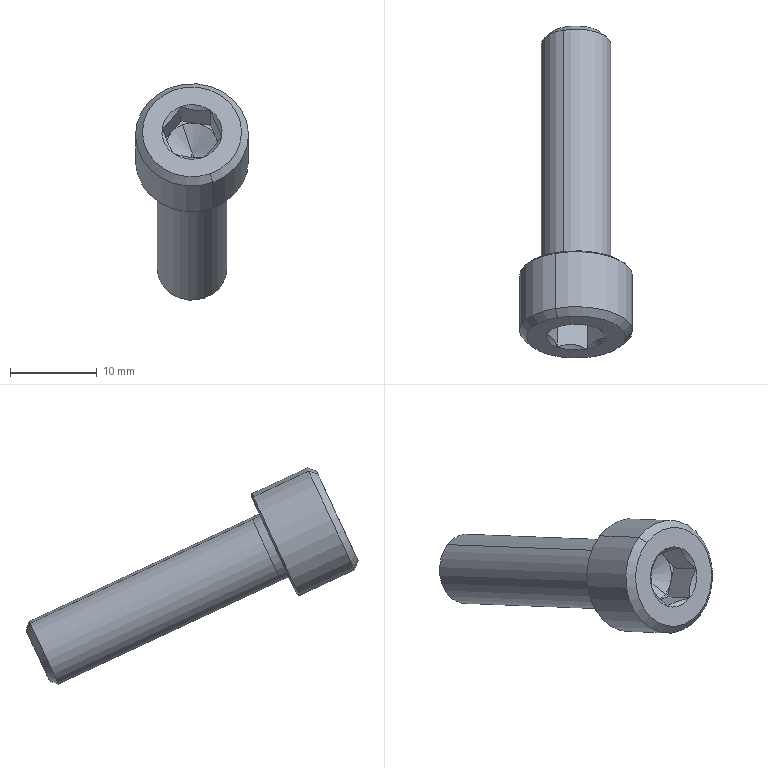Component | SolidWorks | 1369126_DSM_40_270_CC_HD_A_B_0-1_DIN_912_M8x30_F-2 | 1 solid | 35 faces | box 13 x 38.21 x 24.91 mm | volume 2408 mm3 | cone 16 | plane 15 | cylinder 4 | commonest cylinder face diameters 8 x2 13 x2
STEP:
#1=COLOUR_RGB('',0.7922,0.8196,0.9333);
#2=FILL_AREA_STYLE_COLOUR('',#1);
#3=FILL_AREA_STYLE('',(#2));
#4=SURFACE_STYLE_FILL_AREA(#3);
#5=SURFACE_SIDE_STYLE('',(#4));
#6=SURFACE_STYLE_USAGE(.BOTH.,#5);
#7=PRESENTATION_STYLE_ASSIGNMENT((#6));
#8=CARTESIAN_POINT('',(-9.795,80.913,10.266));
#9=VERTEX_POINT('',#8);
#10=CARTESIAN_POINT('',(-9.839,80.898,10.394));
#11=VERTEX_POINT('',#10);
#12=CARTESIAN_POINT('',(-9.839,80.898,10.394));
#13=DIRECTION('',(-0.3195,-0.113,0.9408));
#14=VECTOR('',#13,39.37);
#15=LINE('',#12,#14);
#16=EDGE_CURVE('',#9,#11,#15,.T.);
#17=ORIENTED_EDGE('',*,*,#16,.F.);
#18=CARTESIAN_POINT('',(-9.751,80.805,10.195));
#19=VERTEX_POINT('',#18);
#20=CARTESIAN_POINT('',(-9.751,80.805,10.195));
#21=DIRECTION('',(0.3195,-0.7933,-0.5182));
#22=VECTOR('',#21,39.37);
#23=LINE('',#20,#22);
#24=EDGE_CURVE('',#9,#19,#23,.T.);
#25=ORIENTED_EDGE('',*,*,#24,.T.);
#26=CARTESIAN_POINT('',(-9.702,80.82,10.228));
#27=VERTEX_POINT('',#26);
#28=CARTESIAN_POINT('',(-9.795,80.851,10.295));
#29=DIRECTION('',(0.,-0.9063,0.4226));
#30=DIRECTION('',(-0.3689,0.3928,0.8424));
#31=AXIS2_PLACEMENT_3D('',#28,#29,#30);
#32=CIRCLE('',#31,0.1181);
#33=EDGE_CURVE('',#19,#27,#32,.T.);
#34=ORIENTED_EDGE('',*,*,#33,.T.);
#35=CARTESIAN_POINT('',(-9.685,80.87,10.334));
#36=VERTEX_POINT('',#35);
#37=CARTESIAN_POINT('',(-9.795,80.851,10.295));
#38=DIRECTION('',(0.,-0.9063,0.4226));
#39=DIRECTION('',(-0.3689,0.3928,0.8424));
#40=AXIS2_PLACEMENT_3D('',#37,#38,#39);
#41=CIRCLE('',#40,0.1181);
#42=EDGE_CURVE('',#27,#36,#41,.T.);
#43=ORIENTED_EDGE('',*,*,#42,.T.);
#44=CARTESIAN_POINT('',(-9.778,80.901,10.401));
#45=VERTEX_POINT('',#44);
#46=CARTESIAN_POINT('',(-9.795,80.851,10.295));
#47=DIRECTION('',(0.,-0.9063,0.4226));
#48=DIRECTION('',(-0.3689,0.3928,0.8424));
#49=AXIS2_PLACEMENT_3D('',#46,#47,#48);
#50=CIRCLE('',#49,0.1181);
#51=EDGE_CURVE('',#36,#45,#50,.T.);
#52=ORIENTED_EDGE('',*,*,#51,.T.);
#53=CARTESIAN_POINT('',(-9.795,80.851,10.295));
#54=DIRECTION('',(0.,-0.9063,0.4226));
#55=DIRECTION('',(-0.3689,0.3928,0.8424));
#56=AXIS2_PLACEMENT_3D('',#53,#54,#55);
#57=CIRCLE('',#56,0.1181);
#58=EDGE_CURVE('',#45,#11,#57,.T.);
#59=ORIENTED_EDGE('',*,*,#58,.T.);
#60=EDGE_LOOP('',(#17,#25,#34,#43,#52,#59));
#61=FACE_OUTER_BOUND('',#60,.T.);
#62=CARTESIAN_POINT('',(-9.795,80.851,10.295));
#63=DIRECTION('',(0.,-0.9063,0.4226));
#64=DIRECTION('',(-0.3689,0.3928,0.8424));
#65=AXIS2_PLACEMENT_3D('',#62,#63,#64);
#66=CONICAL_SURFACE('',#65,0.1181,1.047);
#67=ADVANCED_FACE('',(#61),#66,.F.);
#68=CARTESIAN_POINT('',(-9.842,82.114,9.836));
#69=VERTEX_POINT('',#68);
#70=CARTESIAN_POINT('',(-9.748,82.014,9.622));
#71=VERTEX_POINT('',#70);
#72=CARTESIAN_POINT('',(-9.795,82.064,9.729));
#73=DIRECTION('',(0.,-0.9063,0.4226));
#74=DIRECTION('',(-0.3689,0.3928,0.8424));
#75=AXIS2_PLACEMENT_3D('',#72,#73,#74);
#76=CIRCLE('',#75,0.1273);
#77=EDGE_CURVE('',#69,#71,#76,.T.);
#78=ORIENTED_EDGE('',*,*,#77,.T.);
#79=CARTESIAN_POINT('',(-9.737,81.975,9.609));
#80=VERTEX_POINT('',#79);
#81=CARTESIAN_POINT('',(-9.748,82.014,9.622));
#82=DIRECTION('',(0.2609,-0.9186,-0.2968));
#83=VECTOR('',#82,39.37);
#84=LINE('',#81,#83);
#85=EDGE_CURVE('',#71,#80,#84,.T.);
#86=ORIENTED_EDGE('',*,*,#85,.T.);
#87=CARTESIAN_POINT('',(-9.853,82.099,9.874));
#88=VERTEX_POINT('',#87);
#89=CARTESIAN_POINT('',(-9.795,82.037,9.742));
#90=DIRECTION('',(0.,-0.9063,0.4226));
#91=DIRECTION('',(-0.3689,0.3928,0.8424));
#92=AXIS2_PLACEMENT_3D('',#89,#90,#91);
#93=CIRCLE('',#92,0.1575);
#94=EDGE_CURVE('',#88,#80,#93,.T.);
#95=ORIENTED_EDGE('',*,*,#94,.F.);
#96=CARTESIAN_POINT('',(-9.842,82.114,9.836));
#97=DIRECTION('',(-0.2609,-0.3631,0.8945));
#98=VECTOR('',#97,39.37);
#99=LINE('',#96,#98);
#100=EDGE_CURVE('',#69,#88,#99,.T.);
#101=ORIENTED_EDGE('',*,*,#100,.F.);
#102=EDGE_LOOP('',(#78,#86,#95,#101));
#103=FACE_OUTER_BOUND('',#102,.T.);
#104=CARTESIAN_POINT('',(-9.795,82.064,9.729));
#105=DIRECTION('',(0.,-0.9063,0.4226));
#106=DIRECTION('',(-0.3689,0.3928,0.8424));
#107=AXIS2_PLACEMENT_3D('',#104,#105,#106);
#108=CONICAL_SURFACE('',#107,0.1273,0.7854);
#109=ADVANCED_FACE('',(#103),#108,.T.);
#110=ORIENTED_EDGE('',*,*,#94,.T.);
#111=CARTESIAN_POINT('',(-9.737,80.968,10.079));
#112=VERTEX_POINT('',#111);
#113=CARTESIAN_POINT('',(-9.737,82.003,9.596));
#114=DIRECTION('',(0.,-0.9063,0.4226));
#115=VECTOR('',#114,39.37);
#116=LINE('',#113,#115);
#117=EDGE_CURVE('',#80,#112,#116,.T.);
#118=ORIENTED_EDGE('',*,*,#117,.T.);
#119=CARTESIAN_POINT('',(-9.853,81.092,10.344));
#120=VERTEX_POINT('',#119);
#121=CARTESIAN_POINT('',(-9.795,81.03,10.211));
#122=DIRECTION('',(0.,-0.9063,0.4226));
#123=DIRECTION('',(-0.3689,0.3928,0.8424));
#124=AXIS2_PLACEMENT_3D('',#121,#122,#123);
#125=CIRCLE('',#124,0.1575);
#126=EDGE_CURVE('',#120,#112,#125,.T.);
#127=ORIENTED_EDGE('',*,*,#126,.F.);
#128=CARTESIAN_POINT('',(-9.853,82.126,9.862));
#129=DIRECTION('',(0.,-0.9063,0.4226));
#130=VECTOR('',#129,39.37);
#131=LINE('',#128,#130);
#132=EDGE_CURVE('',#88,#120,#131,.T.);
#133=ORIENTED_EDGE('',*,*,#132,.F.);
#134=EDGE_LOOP('',(#110,#118,#127,#133));
#135=FACE_OUTER_BOUND('',#134,.T.);
#136=CARTESIAN_POINT('',(-9.795,82.064,9.729));
#137=DIRECTION('',(0.,-0.9063,0.4226));
#138=DIRECTION('',(-0.3689,0.3928,0.8424));
#139=AXIS2_PLACEMENT_3D('',#136,#137,#138);
#140=CYLINDRICAL_SURFACE('',#139,0.1575);
#141=ADVANCED_FACE('',(#135),#140,.T.);
#142=ORIENTED_EDGE('',*,*,#126,.T.);
#143=CARTESIAN_POINT('',(-9.736,80.931,10.094));
#144=VERTEX_POINT('',#143);
#145=CARTESIAN_POINT('',(-9.737,80.968,10.079));
#146=DIRECTION('',(0.01806,-0.9245,0.3809));
#147=VECTOR('',#146,39.37);
#148=LINE('',#145,#147);
#149=EDGE_CURVE('',#112,#144,#148,.T.);
#150=ORIENTED_EDGE('',*,*,#149,.T.);
#151=CARTESIAN_POINT('',(-9.854,81.057,10.362));
#152=VERTEX_POINT('',#151);
#153=CARTESIAN_POINT('',(-9.795,80.994,10.228));
#154=DIRECTION('',(0.,-0.9063,0.4226));
#155=DIRECTION('',(-0.3689,0.3928,0.8424));
#156=AXIS2_PLACEMENT_3D('',#153,#154,#155);
#157=CIRCLE('',#156,0.1594);
#158=EDGE_CURVE('',#152,#144,#157,.T.);
#159=ORIENTED_EDGE('',*,*,#158,.F.);
#160=CARTESIAN_POINT('',(-9.853,81.092,10.344));
#161=DIRECTION('',(-0.01806,-0.886,0.4634));
#162=VECTOR('',#161,39.37);
#163=LINE('',#160,#162);
#164=EDGE_CURVE('',#120,#152,#163,.T.);
#165=ORIENTED_EDGE('',*,*,#164,.F.);
#166=EDGE_LOOP('',(#142,#150,#159,#165));
#167=FACE_OUTER_BOUND('',#166,.T.);
#168=CARTESIAN_POINT('',(-9.795,81.03,10.211));
#169=DIRECTION('',(0.,-0.9063,0.4226));
#170=DIRECTION('',(-0.3689,0.3928,0.8424));
#171=AXIS2_PLACEMENT_3D('',#168,#169,#170);
#172=CONICAL_SURFACE('',#171,0.1575,0.04898);
#173=ADVANCED_FACE('',(#167),#172,.T.);
#174=CARTESIAN_POINT('',(-9.887,81.091,10.437));
#175=VERTEX_POINT('',#174);
#176=CARTESIAN_POINT('',(-9.703,80.896,10.019));
#177=VERTEX_POINT('',#176);
#178=CARTESIAN_POINT('',(-9.795,80.994,10.228));
#179=DIRECTION('',(0.,-0.9063,0.4226));
#180=DIRECTION('',(-0.3689,0.3928,0.8424));
#181=AXIS2_PLACEMENT_3D('',#178,#179,#180);
#182=CIRCLE('',#181,0.248);
#183=EDGE_CURVE('',#175,#177,#182,.T.);
#184=ORIENTED_EDGE('',*,*,#183,.T.);
#185=CARTESIAN_POINT('',(-9.701,80.886,10.016));
#186=VERTEX_POINT('',#185);
#187=CARTESIAN_POINT('',(-9.703,80.896,10.019));
#188=DIRECTION('',(0.2609,-0.9186,-0.2968));
#189=VECTOR('',#188,39.37);
#190=LINE('',#187,#189);
#191=EDGE_CURVE('',#177,#186,#190,.T.);
#192=ORIENTED_EDGE('',*,*,#191,.T.);
#193=CARTESIAN_POINT('',(-9.889,81.087,10.447));
#194=VERTEX_POINT('',#193);
#195=CARTESIAN_POINT('',(-9.795,80.987,10.232));
#196=DIRECTION('',(0.,-0.9063,0.4226));
#197=DIRECTION('',(-0.3689,0.3928,0.8424));
#198=AXIS2_PLACEMENT_3D('',#195,#196,#197);
#199=CIRCLE('',#198,0.2559);
#200=EDGE_CURVE('',#194,#186,#199,.T.);
#201=ORIENTED_EDGE('',*,*,#200,.F.);
#202=CARTESIAN_POINT('',(-9.887,81.091,10.437));
#203=DIRECTION('',(-0.2609,-0.3631,0.8945));
#204=VECTOR('',#203,39.37);
#205=LINE('',#202,#204);
#206=EDGE_CURVE('',#175,#194,#205,.T.);
#207=ORIENTED_EDGE('',*,*,#206,.F.);
#208=EDGE_LOOP('',(#184,#192,#201,#207));
#209=FACE_OUTER_BOUND('',#208,.T.);
#210=CARTESIAN_POINT('',(-9.795,80.994,10.228));
#211=DIRECTION('',(0.,-0.9063,0.4226));
#212=DIRECTION('',(-0.3689,0.3928,0.8424));
#213=AXIS2_PLACEMENT_3D('',#210,#211,#212);
#214=CONICAL_SURFACE('',#213,0.248,0.7854);
#215=ADVANCED_FACE('',(#209),#214,.T.);
#216=ORIENTED_EDGE('',*,*,#200,.T.);
#217=CARTESIAN_POINT('',(-9.701,80.636,10.132));
#218=VERTEX_POINT('',#217);
#219=CARTESIAN_POINT('',(-9.701,81.964,9.513));
#220=DIRECTION('',(0.,-0.9063,0.4226));
#221=VECTOR('',#220,39.37);
#222=LINE('',#219,#221);
#223=EDGE_CURVE('',#186,#218,#222,.T.);
#224=ORIENTED_EDGE('',*,*,#223,.T.);
#225=CARTESIAN_POINT('',(-9.889,80.838,10.564));
#226=VERTEX_POINT('',#225);
#227=CARTESIAN_POINT('',(-9.795,80.737,10.348));
#228=DIRECTION('',(0.,-0.9063,0.4226));
#229=DIRECTION('',(-0.3689,0.3928,0.8424));
#230=AXIS2_PLACEMENT_3D('',#227,#228,#229);
#231=CIRCLE('',#230,0.2559);
#232=EDGE_CURVE('',#226,#218,#231,.T.);
#233=ORIENTED_EDGE('',*,*,#232,.F.);
#234=CARTESIAN_POINT('',(-9.889,82.165,9.945));
#235=DIRECTION('',(0.,-0.9063,0.4226));
#236=VECTOR('',#235,39.37);
#237=LINE('',#234,#236);
#238=EDGE_CURVE('',#194,#226,#237,.T.);
#239=ORIENTED_EDGE('',*,*,#238,.F.);
#240=EDGE_LOOP('',(#216,#224,#233,#239));
#241=FACE_OUTER_BOUND('',#240,.T.);
#242=CARTESIAN_POINT('',(-9.795,82.064,9.729));
#243=DIRECTION('',(0.,-0.9063,0.4226));
#244=DIRECTION('',(-0.3689,0.3928,0.8424));
#245=AXIS2_PLACEMENT_3D('',#242,#243,#244);
#246=CYLINDRICAL_SURFACE('',#245,0.2559);
#247=ADVANCED_FACE('',(#241),#246,.T.);
#248=CARTESIAN_POINT('',(-9.878,80.797,10.55));
#249=VERTEX_POINT('',#248);
#250=CARTESIAN_POINT('',(-9.712,80.62,10.172));
#251=VERTEX_POINT('',#250);
#252=CARTESIAN_POINT('',(-9.795,80.708,10.361));
#253=DIRECTION('',(0.,-0.9063,0.4226));
#254=DIRECTION('',(-0.3689,0.3928,0.8424));
#255=AXIS2_PLACEMENT_3D('',#252,#253,#254);
#256=CIRCLE('',#255,0.2244);
#257=EDGE_CURVE('',#249,#251,#256,.T.);
#258=ORIENTED_EDGE('',*,*,#257,.F.);
#259=CARTESIAN_POINT('',(-9.889,80.838,10.564));
#260=DIRECTION('',(-0.2609,0.9186,0.2968));
#261=VECTOR('',#260,39.37);
#262=LINE('',#259,#261);
#263=EDGE_CURVE('',#249,#226,#262,.T.);
#264=ORIENTED_EDGE('',*,*,#263,.T.);
#265=ORIENTED_EDGE('',*,*,#232,.T.);
#266=CARTESIAN_POINT('',(-9.701,80.636,10.132));
#267=DIRECTION('',(0.2609,0.3631,-0.8945));
#268=VECTOR('',#267,39.37);
#269=LINE('',#266,#268);
#270=EDGE_CURVE('',#251,#218,#269,.T.);
#271=ORIENTED_EDGE('',*,*,#270,.F.);
#272=EDGE_LOOP('',(#258,#264,#265,#271));
#273=FACE_OUTER_BOUND('',#272,.T.);
#274=CARTESIAN_POINT('',(-9.795,80.737,10.348));
#275=DIRECTION('',(-0.,0.9063,-0.4226));
#276=DIRECTION('',(0.3689,-0.3928,-0.8424));
#277=AXIS2_PLACEMENT_3D('',#274,#275,#276);
#278=CONICAL_SURFACE('',#277,0.2559,0.7854);
#279=ADVANCED_FACE('',(#273),#278,.T.);
#280=CARTESIAN_POINT('',(-9.745,80.655,10.246));
#281=VERTEX_POINT('',#280);
#282=CARTESIAN_POINT('',(-9.66,80.7,10.343));
#283=VERTEX_POINT('',#282);
#284=CARTESIAN_POINT('',(-9.795,80.708,10.361));
#285=DIRECTION('',(0.,-0.9063,0.4226));
#286=DIRECTION('',(-0.3689,0.3928,0.8424));
#287=AXIS2_PLACEMENT_3D('',#284,#285,#286);
#288=CIRCLE('',#287,0.1364);
#289=EDGE_CURVE('',#281,#283,#288,.T.);
#290=ORIENTED_EDGE('',*,*,#289,.T.);
#291=CARTESIAN_POINT('',(-9.66,80.7,10.343));
#292=CARTESIAN_POINT('',(-9.667,80.701,10.334));
#293=CARTESIAN_POINT('',(-9.673,80.702,10.324));
#294=CARTESIAN_POINT('',(-9.684,80.701,10.31));
#295=CARTESIAN_POINT('',(-9.688,80.7,10.305));
#296=CARTESIAN_POINT('',(-9.695,80.698,10.296));
#297=CARTESIAN_POINT('',(-9.699,80.696,10.292));
#298=CARTESIAN_POINT('',(-9.71,80.69,10.279));
#299=CARTESIAN_POINT('',(-9.717,80.685,10.271));
#300=CARTESIAN_POINT('',(-9.731,80.671,10.258));
#301=CARTESIAN_POINT('',(-9.738,80.663,10.252));
#302=CARTESIAN_POINT('',(-9.745,80.655,10.246));
#303=B_SPLINE_CURVE_WITH_KNOTS('',3,(#291,#292,#293,#294,#295,#296,#297,#298,#299,#300,#301,#302),.UNSPECIFIED.,.F.,.F.,(4,2,2,2,2,4),(0.00000025,0.0008948,0.001342,0.001789,0.002684,0.003579),.UNSPECIFIED.);
#304=EDGE_CURVE('',#283,#281,#303,.T.);
#305=ORIENTED_EDGE('',*,*,#304,.T.);
#306=EDGE_LOOP('',(#290,#305));
#307=FACE_OUTER_BOUND('',#306,.T.);
#308=CARTESIAN_POINT('',(-9.795,80.708,10.361));
#309=DIRECTION('',(0.,-0.9063,0.4226));
#310=DIRECTION('',(-0.3689,0.3928,0.8424));
#311=AXIS2_PLACEMENT_3D('',#308,#309,#310);
#312=CONICAL_SURFACE('',#311,0.1364,0.7854);
#313=ADVANCED_FACE('',(#307),#312,.F.);
#314=CARTESIAN_POINT('',(-9.88,80.663,10.264));
#315=VERTEX_POINT('',#314);
#316=CARTESIAN_POINT('',(-9.795,80.708,10.361));
#317=DIRECTION('',(0.,-0.9063,0.4226));
#318=DIRECTION('',(-0.3689,0.3928,0.8424));
#319=AXIS2_PLACEMENT_3D('',#316,#317,#318);
#320=CIRCLE('',#319,0.1364);
#321=EDGE_CURVE('',#315,#281,#320,.T.);
#322=ORIENTED_EDGE('',*,*,#321,.T.);
#323=CARTESIAN_POINT('',(-9.745,80.655,10.246));
#324=CARTESIAN_POINT('',(-9.755,80.66,10.246));
#325=CARTESIAN_POINT('',(-9.766,80.665,10.245));
#326=CARTESIAN_POINT('',(-9.783,80.671,10.245));
#327=CARTESIAN_POINT('',(-9.788,80.672,10.245));
#328=CARTESIAN_POINT('',(-9.8,80.674,10.246));
#329=CARTESIAN_POINT('',(-9.806,80.675,10.247));
#330=CARTESIAN_POINT('',(-9.824,80.676,10.249));
#331=CARTESIAN_POINT('',(-9.835,80.675,10.251));
#332=CARTESIAN_POINT('',(-9.858,80.671,10.257));
#333=CARTESIAN_POINT('',(-9.869,80.667,10.261));
#334=CARTESIAN_POINT('',(-9.88,80.663,10.264));
#335=B_SPLINE_CURVE_WITH_KNOTS('',3,(#323,#324,#325,#326,#327,#328,#329,#330,#331,#332,#333,#334),.UNSPECIFIED.,.F.,.F.,(4,2,2,2,2,4),(0.00000025,0.0008948,0.001342,0.001789,0.002684,0.003579),.UNSPECIFIED.);
#336=EDGE_CURVE('',#281,#315,#335,.T.);
#337=ORIENTED_EDGE('',*,*,#336,.T.);
#338=EDGE_LOOP('',(#322,#337));
#339=FACE_OUTER_BOUND('',#338,.T.);
#340=CARTESIAN_POINT('',(-9.795,80.708,10.361));
#341=DIRECTION('',(0.,-0.9063,0.4226));
#342=DIRECTION('',(-0.3689,0.3928,0.8424));
#343=AXIS2_PLACEMENT_3D('',#340,#341,#342);
#344=CONICAL_SURFACE('',#343,0.1364,0.7854);
#345=ADVANCED_FACE('',(#339),#344,.F.);
#346=CARTESIAN_POINT('',(-9.93,80.717,10.379));
#347=VERTEX_POINT('',#346);
#348=CARTESIAN_POINT('',(-9.795,80.708,10.361));
#349=DIRECTION('',(0.,-0.9063,0.4226));
#350=DIRECTION('',(-0.3689,0.3928,0.8424));
#351=AXIS2_PLACEMENT_3D('',#348,#349,#350);
#352=CIRCLE('',#351,0.1364);
#353=EDGE_CURVE('',#347,#315,#352,.T.);
#354=ORIENTED_EDGE('',*,*,#353,.T.);
#355=CARTESIAN_POINT('',(-9.88,80.663,10.264));
#356=CARTESIAN_POINT('',(-9.884,80.672,10.271));
#357=CARTESIAN_POINT('',(-9.888,80.681,10.278));
#358=CARTESIAN_POINT('',(-9.896,80.696,10.295));
#359=CARTESIAN_POINT('',(-9.9,80.702,10.304));
#360=CARTESIAN_POINT('',(-9.909,80.711,10.324));
#361=CARTESIAN_POINT('',(-9.914,80.714,10.335));
#362=CARTESIAN_POINT('',(-9.92,80.717,10.351));
#363=CARTESIAN_POINT('',(-9.922,80.717,10.357));
#364=CARTESIAN_POINT('',(-9.926,80.717,10.368));
#365=CARTESIAN_POINT('',(-9.928,80.717,10.374));
#366=CARTESIAN_POINT('',(-9.93,80.717,10.379));
#367=B_SPLINE_CURVE_WITH_KNOTS('',3,(#355,#356,#357,#358,#359,#360,#361,#362,#363,#364,#365,#366),.UNSPECIFIED.,.F.,.F.,(4,2,2,2,2,4),(0.00225,0.003148,0.004045,0.004943,0.005392,0.005841),.UNSPECIFIED.);
#368=EDGE_CURVE('',#315,#347,#367,.T.);
#369=ORIENTED_EDGE('',*,*,#368,.T.);
#370=EDGE_LOOP('',(#354,#369));
#371=FACE_OUTER_BOUND('',#370,.T.);
#372=CARTESIAN_POINT('',(-9.795,80.708,10.361));
#373=DIRECTION('',(0.,-0.9063,0.4226));
#374=DIRECTION('',(-0.3689,0.3928,0.8424));
#375=AXIS2_PLACEMENT_3D('',#372,#373,#374);
#376=CONICAL_SURFACE('',#375,0.1364,0.7854);
#377=ADVANCED_FACE('',(#371),#376,.F.);
#378=CARTESIAN_POINT('',(-9.845,80.762,10.476));
#379=VERTEX_POINT('',#378);
#380=CARTESIAN_POINT('',(-9.795,80.708,10.361));
#381=DIRECTION('',(0.,-0.9063,0.4226));
#382=DIRECTION('',(-0.3689,0.3928,0.8424));
#383=AXIS2_PLACEMENT_3D('',#380,#381,#382);
#384=CIRCLE('',#383,0.1364);
#385=EDGE_CURVE('',#379,#347,#384,.T.);
#386=ORIENTED_EDGE('',*,*,#385,.T.);
#387=CARTESIAN_POINT('',(-9.93,80.717,10.379));
#388=CARTESIAN_POINT('',(-9.923,80.725,10.385));
#389=CARTESIAN_POINT('',(-9.917,80.733,10.39));
#390=CARTESIAN_POINT('',(-9.906,80.743,10.4));
#391=CARTESIAN_POINT('',(-9.903,80.746,10.404));
#392=CARTESIAN_POINT('',(-9.895,80.751,10.411));
#393=CARTESIAN_POINT('',(-9.891,80.754,10.416));
#394=CARTESIAN_POINT('',(-9.88,80.76,10.428));
#395=CARTESIAN_POINT('',(-9.873,80.762,10.437));
#396=CARTESIAN_POINT('',(-9.859,80.764,10.457));
#397=CARTESIAN_POINT('',(-9.852,80.763,10.466));
#398=CARTESIAN_POINT('',(-9.845,80.762,10.476));
#399=B_SPLINE_CURVE_WITH_KNOTS('',3,(#387,#388,#389,#390,#391,#392,#393,#394,#395,#396,#397,#398),.UNSPECIFIED.,.F.,.F.,(4,2,2,2,2,4),(0.00000025,0.0008948,0.001342,0.001789,0.002684,0.003579),.UNSPECIFIED.);
#400=EDGE_CURVE('',#347,#379,#399,.T.);
#401=ORIENTED_EDGE('',*,*,#400,.T.);
#402=EDGE_LOOP('',(#386,#401));
#403=FACE_OUTER_BOUND('',#402,.T.);
#404=CARTESIAN_POINT('',(-9.795,80.708,10.361));
#405=DIRECTION('',(0.,-0.9063,0.4226));
#406=DIRECTION('',(-0.3689,0.3928,0.8424));
#407=AXIS2_PLACEMENT_3D('',#404,#405,#406);
#408=CONICAL_SURFACE('',#407,0.1364,0.7854);
#409=ADVANCED_FACE('',(#403),#408,.F.);
#410=CARTESIAN_POINT('',(-9.71,80.754,10.458));
#411=VERTEX_POINT('',#410);
#412=CARTESIAN_POINT('',(-9.795,80.708,10.361));
#413=DIRECTION('',(0.,-0.9063,0.4226));
#414=DIRECTION('',(-0.3689,0.3928,0.8424));
#415=AXIS2_PLACEMENT_3D('',#412,#413,#414);
#416=CIRCLE('',#415,0.1364);
#417=EDGE_CURVE('',#411,#379,#416,.T.);
#418=ORIENTED_EDGE('',*,*,#417,.T.);
#419=CARTESIAN_POINT('',(-9.845,80.762,10.476));
#420=CARTESIAN_POINT('',(-9.835,80.766,10.473));
#421=CARTESIAN_POINT('',(-9.824,80.77,10.469));
#422=CARTESIAN_POINT('',(-9.807,80.773,10.465));
#423=CARTESIAN_POINT('',(-9.802,80.774,10.464));
#424=CARTESIAN_POINT('',(-9.79,80.775,10.461));
#425=CARTESIAN_POINT('',(-9.784,80.775,10.46));
#426=CARTESIAN_POINT('',(-9.766,80.774,10.458));
#427=CARTESIAN_POINT('',(-9.755,80.771,10.457));
#428=CARTESIAN_POINT('',(-9.732,80.764,10.457));
#429=CARTESIAN_POINT('',(-9.721,80.759,10.457));
#430=CARTESIAN_POINT('',(-9.71,80.754,10.458));
#431=B_SPLINE_CURVE_WITH_KNOTS('',3,(#419,#420,#421,#422,#423,#424,#425,#426,#427,#428,#429,#430),.UNSPECIFIED.,.F.,.F.,(4,2,2,2,2,4),(0.00000025,0.0008948,0.001342,0.001789,0.002684,0.003579),.UNSPECIFIED.);
#432=EDGE_CURVE('',#379,#411,#431,.T.);
#433=ORIENTED_EDGE('',*,*,#432,.T.);
#434=EDGE_LOOP('',(#418,#433));
#435=FACE_OUTER_BOUND('',#434,.T.);
#436=CARTESIAN_POINT('',(-9.795,80.708,10.361));
#437=DIRECTION('',(0.,-0.9063,0.4226));
#438=DIRECTION('',(-0.3689,0.3928,0.8424));
#439=AXIS2_PLACEMENT_3D('',#436,#437,#438);
#440=CONICAL_SURFACE('',#439,0.1364,0.7854);
#441=ADVANCED_FACE('',(#435),#440,.F.);
#442=CARTESIAN_POINT('',(-9.795,80.708,10.361));
#443=DIRECTION('',(0.,-0.9063,0.4226));
#444=DIRECTION('',(-0.3689,0.3928,0.8424));
#445=AXIS2_PLACEMENT_3D('',#442,#443,#444);
#446=CIRCLE('',#445,0.1364);
#447=EDGE_CURVE('',#283,#411,#446,.T.);
#448=ORIENTED_EDGE('',*,*,#447,.T.);
#449=CARTESIAN_POINT('',(-9.71,80.754,10.458));
#450=CARTESIAN_POINT('',(-9.708,80.754,10.453));
#451=CARTESIAN_POINT('',(-9.706,80.754,10.447));
#452=CARTESIAN_POINT('',(-9.702,80.754,10.436));
#453=CARTESIAN_POINT('',(-9.7,80.753,10.43));
#454=CARTESIAN_POINT('',(-9.694,80.751,10.414));
#455=CARTESIAN_POINT('',(-9.69,80.748,10.403));
#456=CARTESIAN_POINT('',(-9.681,80.739,10.383));
#457=CARTESIAN_POINT('',(-9.676,80.732,10.374));
#458=CARTESIAN_POINT('',(-9.668,80.718,10.357));
#459=CARTESIAN_POINT('',(-9.664,80.709,10.35));
#460=CARTESIAN_POINT('',(-9.66,80.7,10.343));
#461=B_SPLINE_CURVE_WITH_KNOTS('',3,(#449,#450,#451,#452,#453,#454,#455,#456,#457,#458,#459,#460),.UNSPECIFIED.,.F.,.F.,(4,2,2,2,2,4),(0.001842,0.00229,0.002739,0.003636,0.004533,0.005431),.UNSPECIFIED.);
#462=EDGE_CURVE('',#411,#283,#461,.T.);
#463=ORIENTED_EDGE('',*,*,#462,.T.);
#464=EDGE_LOOP('',(#448,#463));
#465=FACE_OUTER_BOUND('',#464,.T.);
#466=CARTESIAN_POINT('',(-9.795,80.708,10.361));
#467=DIRECTION('',(0.,-0.9063,0.4226));
#468=DIRECTION('',(-0.3689,0.3928,0.8424));
#469=AXIS2_PLACEMENT_3D('',#466,#467,#468);
#470=CONICAL_SURFACE('',#469,0.1364,0.7854);
#471=ADVANCED_FACE('',(#465),#470,.F.);
#472=ORIENTED_EDGE('',*,*,#385,.F.);
#473=ORIENTED_EDGE('',*,*,#417,.F.);
#474=ORIENTED_EDGE('',*,*,#447,.F.);
#475=ORIENTED_EDGE('',*,*,#289,.F.);
#476=ORIENTED_EDGE('',*,*,#321,.F.);
#477=ORIENTED_EDGE('',*,*,#353,.F.);
#478=EDGE_LOOP('',(#472,#473,#474,#475,#476,#477));
#479=FACE_BOUND('',#478,.T.);
#480=CARTESIAN_POINT('',(-9.795,80.708,10.361));
#481=DIRECTION('',(0.,-0.9063,0.4226));
#482=DIRECTION('',(-0.3689,0.3928,0.8424));
#483=AXIS2_PLACEMENT_3D('',#480,#481,#482);
#484=CIRCLE('',#483,0.2244);
#485=EDGE_CURVE('',#251,#249,#484,.T.);
#486=ORIENTED_EDGE('',*,*,#485,.T.);
#487=ORIENTED_EDGE('',*,*,#257,.T.);
#488=EDGE_LOOP('',(#486,#487));
#489=FACE_OUTER_BOUND('',#488,.T.);
#490=CARTESIAN_POINT('',(-9.922,80.687,10.316));
#491=DIRECTION('',(-0.,0.9063,-0.4226));
#492=DIRECTION('',(0.3689,-0.3928,-0.8424));
#493=AXIS2_PLACEMENT_3D('',#490,#491,#492);
#494=PLANE('',#493);
#495=ADVANCED_FACE('',(#479,#489),#494,.F.);
#496=ORIENTED_EDGE('',*,*,#263,.F.);
#497=ORIENTED_EDGE('',*,*,#485,.F.);
#498=ORIENTED_EDGE('',*,*,#270,.T.);
#499=CARTESIAN_POINT('',(-9.795,80.737,10.348));
#500=DIRECTION('',(0.,-0.9063,0.4226));
#501=DIRECTION('',(-0.3689,0.3928,0.8424));
#502=AXIS2_PLACEMENT_3D('',#499,#500,#501);
#503=CIRCLE('',#502,0.2559);
#504=EDGE_CURVE('',#218,#226,#503,.T.);
#505=ORIENTED_EDGE('',*,*,#504,.T.);
#506=EDGE_LOOP('',(#496,#497,#498,#505));
#507=FACE_OUTER_BOUND('',#506,.T.);
#508=CARTESIAN_POINT('',(-9.795,80.737,10.348));
#509=DIRECTION('',(-0.,0.9063,-0.4226));
#510=DIRECTION('',(0.3689,-0.3928,-0.8424));
#511=AXIS2_PLACEMENT_3D('',#508,#509,#510);
#512=CONICAL_SURFACE('',#511,0.2559,0.7854);
#513=ADVANCED_FACE('',(#507),#512,.T.);
#514=ORIENTED_EDGE('',*,*,#223,.F.);
#515=CARTESIAN_POINT('',(-9.795,80.987,10.232));
#516=DIRECTION('',(0.,-0.9063,0.4226));
#517=DIRECTION('',(-0.3689,0.3928,0.8424));
#518=AXIS2_PLACEMENT_3D('',#515,#516,#517);
#519=CIRCLE('',#518,0.2559);
#520=EDGE_CURVE('',#186,#194,#519,.T.);
#521=ORIENTED_EDGE('',*,*,#520,.T.);
#522=ORIENTED_EDGE('',*,*,#238,.T.);
#523=ORIENTED_EDGE('',*,*,#504,.F.);
#524=EDGE_LOOP('',(#514,#521,#522,#523));
#525=FACE_OUTER_BOUND('',#524,.T.);
#526=CARTESIAN_POINT('',(-9.795,82.064,9.729));
#527=DIRECTION('',(0.,-0.9063,0.4226));
#528=DIRECTION('',(-0.3689,0.3928,0.8424));
#529=AXIS2_PLACEMENT_3D('',#526,#527,#528);
#530=CYLINDRICAL_SURFACE('',#529,0.2559);
#531=ADVANCED_FACE('',(#525),#530,.T.);
#532=ORIENTED_EDGE('',*,*,#191,.F.);
#533=CARTESIAN_POINT('',(-9.795,80.994,10.228));
#534=DIRECTION('',(0.,-0.9063,0.4226));
#535=DIRECTION('',(-0.3689,0.3928,0.8424));
#536=AXIS2_PLACEMENT_3D('',#533,#534,#535);
#537=CIRCLE('',#536,0.248);
#538=EDGE_CURVE('',#177,#175,#537,.T.);
#539=ORIENTED_EDGE('',*,*,#538,.T.);
#540=ORIENTED_EDGE('',*,*,#206,.T.);
#541=ORIENTED_EDGE('',*,*,#520,.F.);
#542=EDGE_LOOP('',(#532,#539,#540,#541));
#543=FACE_OUTER_BOUND('',#542,.T.);
#544=CARTESIAN_POINT('',(-9.795,80.994,10.228));
#545=DIRECTION('',(0.,-0.9063,0.4226));
#546=DIRECTION('',(-0.3689,0.3928,0.8424));
#547=AXIS2_PLACEMENT_3D('',#544,#545,#546);
#548=CONICAL_SURFACE('',#547,0.248,0.7854);
#549=ADVANCED_FACE('',(#543),#548,.T.);
#550=ORIENTED_EDGE('',*,*,#183,.F.);
#551=ORIENTED_EDGE('',*,*,#538,.F.);
#552=EDGE_LOOP('',(#550,#551));
#553=FACE_OUTER_BOUND('',#552,.T.);
#554=ORIENTED_EDGE('',*,*,#158,.T.);
#555=CARTESIAN_POINT('',(-9.795,80.994,10.228));
#556=DIRECTION('',(0.,-0.9063,0.4226));
#557=DIRECTION('',(-0.3689,0.3928,0.8424));
#558=AXIS2_PLACEMENT_3D('',#555,#556,#557);
#559=CIRCLE('',#558,0.1594);
#560=EDGE_CURVE('',#144,#152,#559,.T.);
#561=ORIENTED_EDGE('',*,*,#560,.T.);
#562=EDGE_LOOP('',(#554,#561));
#563=FACE_BOUND('',#562,.T.);
#564=CARTESIAN_POINT('',(-10.026,80.955,10.145));
#565=DIRECTION('',(0.,-0.9063,0.4226));
#566=DIRECTION('',(-0.3689,0.3928,0.8424));
#567=AXIS2_PLACEMENT_3D('',#564,#565,#566);
#568=PLANE('',#567);
#569=ADVANCED_FACE('',(#553,#563),#568,.F.);
#570=ORIENTED_EDGE('',*,*,#149,.F.);
#571=CARTESIAN_POINT('',(-9.795,81.03,10.211));
#572=DIRECTION('',(0.,-0.9063,0.4226));
#573=DIRECTION('',(-0.3689,0.3928,0.8424));
#574=AXIS2_PLACEMENT_3D('',#571,#572,#573);
#575=CIRCLE('',#574,0.1575);
#576=EDGE_CURVE('',#112,#120,#575,.T.);
#577=ORIENTED_EDGE('',*,*,#576,.T.);
#578=ORIENTED_EDGE('',*,*,#164,.T.);
#579=ORIENTED_EDGE('',*,*,#560,.F.);
#580=EDGE_LOOP('',(#570,#577,#578,#579));
#581=FACE_OUTER_BOUND('',#580,.T.);
#582=CARTESIAN_POINT('',(-9.795,81.03,10.211));
#583=DIRECTION('',(0.,-0.9063,0.4226));
#584=DIRECTION('',(-0.3689,0.3928,0.8424));
#585=AXIS2_PLACEMENT_3D('',#582,#583,#584);
#586=CONICAL_SURFACE('',#585,0.1575,0.04898);
#587=ADVANCED_FACE('',(#581),#586,.T.);
#588=ORIENTED_EDGE('',*,*,#117,.F.);
#589=CARTESIAN_POINT('',(-9.795,82.037,9.742));
#590=DIRECTION('',(0.,-0.9063,0.4226));
#591=DIRECTION('',(-0.3689,0.3928,0.8424));
#592=AXIS2_PLACEMENT_3D('',#589,#590,#591);
#593=CIRCLE('',#592,0.1575);
#594=EDGE_CURVE('',#80,#88,#593,.T.);
#595=ORIENTED_EDGE('',*,*,#594,.T.);
#596=ORIENTED_EDGE('',*,*,#132,.T.);
#597=ORIENTED_EDGE('',*,*,#576,.F.);
#598=EDGE_LOOP('',(#588,#595,#596,#597));
#599=FACE_OUTER_BOUND('',#598,.T.);
#600=CARTESIAN_POINT('',(-9.795,82.064,9.729));
#601=DIRECTION('',(0.,-0.9063,0.4226));
#602=DIRECTION('',(-0.3689,0.3928,0.8424));
#603=AXIS2_PLACEMENT_3D('',#600,#601,#602);
#604=CYLINDRICAL_SURFACE('',#603,0.1575);
#605=ADVANCED_FACE('',(#599),#604,.T.);
#606=ORIENTED_EDGE('',*,*,#85,.F.);
#607=CARTESIAN_POINT('',(-9.795,82.064,9.729));
#608=DIRECTION('',(0.,-0.9063,0.4226));
#609=DIRECTION('',(-0.3689,0.3928,0.8424));
#610=AXIS2_PLACEMENT_3D('',#607,#608,#609);
#611=CIRCLE('',#610,0.1273);
#612=EDGE_CURVE('',#71,#69,#611,.T.);
#613=ORIENTED_EDGE('',*,*,#612,.T.);
#614=ORIENTED_EDGE('',*,*,#100,.T.);
#615=ORIENTED_EDGE('',*,*,#594,.F.);
#616=EDGE_LOOP('',(#606,#613,#614,#615));
#617=FACE_OUTER_BOUND('',#616,.T.);
#618=CARTESIAN_POINT('',(-9.795,82.064,9.729));
#619=DIRECTION('',(0.,-0.9063,0.4226));
#620=DIRECTION('',(-0.3689,0.3928,0.8424));
#621=AXIS2_PLACEMENT_3D('',#618,#619,#620);
#622=CONICAL_SURFACE('',#621,0.1273,0.7854);
#623=ADVANCED_FACE('',(#617),#622,.T.);
#624=ORIENTED_EDGE('',*,*,#77,.F.);
#625=ORIENTED_EDGE('',*,*,#612,.F.);
#626=EDGE_LOOP('',(#624,#625));
#627=FACE_OUTER_BOUND('',#626,.T.);
#628=CARTESIAN_POINT('',(-9.913,82.045,9.686));
#629=DIRECTION('',(0.,-0.9063,0.4226));
#630=DIRECTION('',(-0.3689,0.3928,0.8424));
#631=AXIS2_PLACEMENT_3D('',#628,#629,#630);
#632=PLANE('',#631);
#633=ADVANCED_FACE('',(#627),#632,.F.);
#634=ORIENTED_EDGE('',*,*,#51,.F.);
#635=CARTESIAN_POINT('',(-9.71,80.896,10.392));
#636=VERTEX_POINT('',#635);
#637=CARTESIAN_POINT('',(-9.66,80.843,10.277));
#638=DIRECTION('',(-0.3689,0.3928,0.8424));
#639=VECTOR('',#638,39.37);
#640=LINE('',#637,#639);
#641=EDGE_CURVE('',#36,#636,#640,.T.);
#642=ORIENTED_EDGE('',*,*,#641,.T.);
#643=CARTESIAN_POINT('',(-9.71,80.896,10.392));
#644=DIRECTION('',(-0.9894,0.06137,0.1316));
#645=VECTOR('',#644,39.37);
#646=LINE('',#643,#645);
#647=EDGE_CURVE('',#636,#45,#646,.T.);
#648=ORIENTED_EDGE('',*,*,#647,.T.);
#649=EDGE_LOOP('',(#634,#642,#648));
#650=FACE_OUTER_BOUND('',#649,.T.);
#651=CARTESIAN_POINT('',(-9.795,80.851,10.295));
#652=DIRECTION('',(0.,-0.9063,0.4226));
#653=DIRECTION('',(-0.3689,0.3928,0.8424));
#654=AXIS2_PLACEMENT_3D('',#651,#652,#653);
#655=PLANE('',#654);
#656=ADVANCED_FACE('',(#650),#655,.T.);
#657=ORIENTED_EDGE('',*,*,#42,.F.);
#658=CARTESIAN_POINT('',(-9.66,80.843,10.277));
#659=VERTEX_POINT('',#658);
#660=CARTESIAN_POINT('',(-9.745,80.798,10.18));
#661=DIRECTION('',(0.6205,0.3314,0.7108));
#662=VECTOR('',#661,39.37);
#663=LINE('',#660,#662);
#664=EDGE_CURVE('',#27,#659,#663,.T.);
#665=ORIENTED_EDGE('',*,*,#664,.T.);
#666=CARTESIAN_POINT('',(-9.66,80.843,10.277));
#667=DIRECTION('',(-0.3689,0.3928,0.8424));
#668=VECTOR('',#667,39.37);
#669=LINE('',#666,#668);
#670=EDGE_CURVE('',#659,#36,#669,.T.);
#671=ORIENTED_EDGE('',*,*,#670,.T.);
#672=EDGE_LOOP('',(#657,#665,#671));
#673=FACE_OUTER_BOUND('',#672,.T.);
#674=CARTESIAN_POINT('',(-9.795,80.851,10.295));
#675=DIRECTION('',(0.,-0.9063,0.4226));
#676=DIRECTION('',(-0.3689,0.3928,0.8424));
#677=AXIS2_PLACEMENT_3D('',#674,#675,#676);
#678=PLANE('',#677);
#679=ADVANCED_FACE('',(#673),#678,.T.);
#680=CARTESIAN_POINT('',(-9.812,80.802,10.189));
#681=VERTEX_POINT('',#680);
#682=CARTESIAN_POINT('',(-9.795,80.851,10.295));
#683=DIRECTION('',(0.,-0.9063,0.4226));
#684=DIRECTION('',(-0.3689,0.3928,0.8424));
#685=AXIS2_PLACEMENT_3D('',#682,#683,#684);
#686=CIRCLE('',#685,0.1181);
#687=EDGE_CURVE('',#681,#19,#686,.T.);
#688=ORIENTED_EDGE('',*,*,#687,.F.);
#689=CARTESIAN_POINT('',(-9.745,80.798,10.18));
#690=VERTEX_POINT('',#689);
#691=CARTESIAN_POINT('',(-9.88,80.806,10.198));
#692=DIRECTION('',(0.9894,-0.06137,-0.1316));
#693=VECTOR('',#692,39.37);
#694=LINE('',#691,#693);
#695=EDGE_CURVE('',#681,#690,#694,.T.);
#696=ORIENTED_EDGE('',*,*,#695,.T.);
#697=CARTESIAN_POINT('',(-9.745,80.798,10.18));
#698=DIRECTION('',(0.6205,0.3314,0.7108));
#699=VECTOR('',#698,39.37);
#700=LINE('',#697,#699);
#701=EDGE_CURVE('',#690,#27,#700,.T.);
#702=ORIENTED_EDGE('',*,*,#701,.T.);
#703=ORIENTED_EDGE('',*,*,#33,.F.);
#704=EDGE_LOOP('',(#688,#696,#702,#703));
#705=FACE_OUTER_BOUND('',#704,.T.);
#706=CARTESIAN_POINT('',(-9.795,80.851,10.295));
#707=DIRECTION('',(0.,-0.9063,0.4226));
#708=DIRECTION('',(-0.3689,0.3928,0.8424));
#709=AXIS2_PLACEMENT_3D('',#706,#707,#708);
#710=PLANE('',#709);
#711=ADVANCED_FACE('',(#705),#710,.T.);
#712=CARTESIAN_POINT('',(-9.905,80.833,10.255));
#713=VERTEX_POINT('',#712);
#714=CARTESIAN_POINT('',(-9.795,80.851,10.295));
#715=DIRECTION('',(0.,-0.9063,0.4226));
#716=DIRECTION('',(-0.3689,0.3928,0.8424));
#717=AXIS2_PLACEMENT_3D('',#714,#715,#716);
#718=CIRCLE('',#717,0.1181);
#719=EDGE_CURVE('',#713,#681,#718,.T.);
#720=ORIENTED_EDGE('',*,*,#719,.F.);
#721=CARTESIAN_POINT('',(-9.88,80.806,10.198));
#722=VERTEX_POINT('',#721);
#723=CARTESIAN_POINT('',(-9.93,80.86,10.313));
#724=DIRECTION('',(0.3689,-0.3928,-0.8424));
#725=VECTOR('',#724,39.37);
#726=LINE('',#723,#725);
#727=EDGE_CURVE('',#713,#722,#726,.T.);
#728=ORIENTED_EDGE('',*,*,#727,.T.);
#729=CARTESIAN_POINT('',(-9.88,80.806,10.198));
#730=DIRECTION('',(0.9894,-0.06137,-0.1316));
#731=VECTOR('',#730,39.37);
#732=LINE('',#729,#731);
#733=EDGE_CURVE('',#722,#681,#732,.T.);
#734=ORIENTED_EDGE('',*,*,#733,.T.);
#735=EDGE_LOOP('',(#720,#728,#734));
#736=FACE_OUTER_BOUND('',#735,.T.);
#737=CARTESIAN_POINT('',(-9.795,80.851,10.295));
#738=DIRECTION('',(0.,-0.9063,0.4226));
#739=DIRECTION('',(-0.3689,0.3928,0.8424));
#740=AXIS2_PLACEMENT_3D('',#737,#738,#739);
#741=PLANE('',#740);
#742=ADVANCED_FACE('',(#736),#741,.T.);
#743=CARTESIAN_POINT('',(-9.888,80.882,10.361));
#744=VERTEX_POINT('',#743);
#745=CARTESIAN_POINT('',(-9.795,80.851,10.295));
#746=DIRECTION('',(0.,-0.9063,0.4226));
#747=DIRECTION('',(-0.3689,0.3928,0.8424));
#748=AXIS2_PLACEMENT_3D('',#745,#746,#747);
#749=CIRCLE('',#748,0.1181);
#750=EDGE_CURVE('',#744,#713,#749,.T.);
#751=ORIENTED_EDGE('',*,*,#750,.F.);
#752=CARTESIAN_POINT('',(-9.93,80.86,10.313));
#753=VERTEX_POINT('',#752);
#754=CARTESIAN_POINT('',(-9.845,80.905,10.41));
#755=DIRECTION('',(-0.6205,-0.3314,-0.7108));
#756=VECTOR('',#755,39.37);
#757=LINE('',#754,#756);
#758=EDGE_CURVE('',#744,#753,#757,.T.);
#759=ORIENTED_EDGE('',*,*,#758,.T.);
#760=CARTESIAN_POINT('',(-9.93,80.86,10.313));
#761=DIRECTION('',(0.3689,-0.3928,-0.8424));
#762=VECTOR('',#761,39.37);
#763=LINE('',#760,#762);
#764=EDGE_CURVE('',#753,#713,#763,.T.);
#765=ORIENTED_EDGE('',*,*,#764,.T.);
#766=EDGE_LOOP('',(#751,#759,#765));
#767=FACE_OUTER_BOUND('',#766,.T.);
#768=CARTESIAN_POINT('',(-9.795,80.851,10.295));
#769=DIRECTION('',(0.,-0.9063,0.4226));
#770=DIRECTION('',(-0.3689,0.3928,0.8424));
#771=AXIS2_PLACEMENT_3D('',#768,#769,#770);
#772=PLANE('',#771);
#773=ADVANCED_FACE('',(#767),#772,.T.);
#774=ORIENTED_EDGE('',*,*,#58,.F.);
#775=CARTESIAN_POINT('',(-9.845,80.905,10.41));
#776=VERTEX_POINT('',#775);
#777=CARTESIAN_POINT('',(-9.71,80.896,10.392));
#778=DIRECTION('',(-0.9894,0.06137,0.1316));
#779=VECTOR('',#778,39.37);
#780=LINE('',#777,#779);
#781=EDGE_CURVE('',#45,#776,#780,.T.);
#782=ORIENTED_EDGE('',*,*,#781,.T.);
#783=CARTESIAN_POINT('',(-9.845,80.905,10.41));
#784=DIRECTION('',(-0.6205,-0.3314,-0.7108));
#785=VECTOR('',#784,39.37);
#786=LINE('',#783,#785);
#787=EDGE_CURVE('',#776,#744,#786,.T.);
#788=ORIENTED_EDGE('',*,*,#787,.T.);
#789=CARTESIAN_POINT('',(-9.795,80.851,10.295));
#790=DIRECTION('',(0.,-0.9063,0.4226));
#791=DIRECTION('',(-0.3689,0.3928,0.8424));
#792=AXIS2_PLACEMENT_3D('',#789,#790,#791);
#793=CIRCLE('',#792,0.1181);
#794=EDGE_CURVE('',#11,#744,#793,.T.);
#795=ORIENTED_EDGE('',*,*,#794,.F.);
#796=EDGE_LOOP('',(#774,#782,#788,#795));
#797=FACE_OUTER_BOUND('',#796,.T.);
#798=CARTESIAN_POINT('',(-9.795,80.851,10.295));
#799=DIRECTION('',(0.,-0.9063,0.4226));
#800=DIRECTION('',(-0.3689,0.3928,0.8424));
#801=AXIS2_PLACEMENT_3D('',#798,#799,#800);
#802=PLANE('',#801);
#803=ADVANCED_FACE('',(#797),#802,.T.);
#804=ORIENTED_EDGE('',*,*,#304,.F.);
#805=CARTESIAN_POINT('',(-9.66,80.843,10.277));
#806=DIRECTION('',(0.,-0.9063,0.4226));
#807=VECTOR('',#806,39.37);
#808=LINE('',#805,#807);
#809=EDGE_CURVE('',#659,#283,#808,.T.);
#810=ORIENTED_EDGE('',*,*,#809,.F.);
#811=ORIENTED_EDGE('',*,*,#664,.F.);
#812=ORIENTED_EDGE('',*,*,#701,.F.);
#813=CARTESIAN_POINT('',(-9.745,80.798,10.18));
#814=DIRECTION('',(0.,-0.9063,0.4226));
#815=VECTOR('',#814,39.37);
#816=LINE('',#813,#815);
#817=EDGE_CURVE('',#690,#281,#816,.T.);
#818=ORIENTED_EDGE('',*,*,#817,.T.);
#819=EDGE_LOOP('',(#804,#810,#811,#812,#818));
#820=FACE_OUTER_BOUND('',#819,.T.);
#821=CARTESIAN_POINT('',(-9.745,80.798,10.18));
#822=DIRECTION('',(0.7842,-0.2622,-0.5623));
#823=DIRECTION('',(0.6205,0.3314,0.7108));
#824=AXIS2_PLACEMENT_3D('',#821,#822,#823);
#825=PLANE('',#824);
#826=ADVANCED_FACE('',(#820),#825,.F.);
#827=ORIENTED_EDGE('',*,*,#336,.F.);
#828=ORIENTED_EDGE('',*,*,#817,.F.);
#829=ORIENTED_EDGE('',*,*,#695,.F.);
#830=ORIENTED_EDGE('',*,*,#733,.F.);
#831=CARTESIAN_POINT('',(-9.88,80.806,10.198));
#832=DIRECTION('',(0.,-0.9063,0.4226));
#833=VECTOR('',#832,39.37);
#834=LINE('',#831,#833);
#835=EDGE_CURVE('',#722,#315,#834,.T.);
#836=ORIENTED_EDGE('',*,*,#835,.T.);
#837=EDGE_LOOP('',(#827,#828,#829,#830,#836));
#838=FACE_OUTER_BOUND('',#837,.T.);
#839=CARTESIAN_POINT('',(-9.88,80.806,10.198));
#840=DIRECTION('',(-0.1452,-0.4181,-0.8967));
#841=DIRECTION('',(0.9894,-0.06137,-0.1316));
#842=AXIS2_PLACEMENT_3D('',#839,#840,#841);
#843=PLANE('',#842);
#844=ADVANCED_FACE('',(#838),#843,.F.);
#845=ORIENTED_EDGE('',*,*,#368,.F.);
#846=ORIENTED_EDGE('',*,*,#835,.F.);
#847=ORIENTED_EDGE('',*,*,#727,.F.);
#848=ORIENTED_EDGE('',*,*,#764,.F.);
#849=CARTESIAN_POINT('',(-9.93,80.86,10.313));
#850=DIRECTION('',(0.,-0.9063,0.4226));
#851=VECTOR('',#850,39.37);
#852=LINE('',#849,#851);
#853=EDGE_CURVE('',#753,#347,#852,.T.);
#854=ORIENTED_EDGE('',*,*,#853,.T.);
#855=EDGE_LOOP('',(#845,#846,#847,#848,#854));
#856=FACE_OUTER_BOUND('',#855,.T.);
#857=CARTESIAN_POINT('',(-9.93,80.86,10.313));
#858=DIRECTION('',(-0.9295,-0.1559,-0.3344));
#859=DIRECTION('',(0.3689,-0.3928,-0.8424));
#860=AXIS2_PLACEMENT_3D('',#857,#858,#859);
#861=PLANE('',#860);
#862=ADVANCED_FACE('',(#856),#861,.F.);
#863=ORIENTED_EDGE('',*,*,#400,.F.);
#864=ORIENTED_EDGE('',*,*,#853,.F.);
#865=ORIENTED_EDGE('',*,*,#758,.F.);
#866=ORIENTED_EDGE('',*,*,#787,.F.);
#867=CARTESIAN_POINT('',(-9.845,80.905,10.41));
#868=DIRECTION('',(0.,-0.9063,0.4226));
#869=VECTOR('',#868,39.37);
#870=LINE('',#867,#869);
#871=EDGE_CURVE('',#776,#379,#870,.T.);
#872=ORIENTED_EDGE('',*,*,#871,.T.);
#873=EDGE_LOOP('',(#863,#864,#865,#866,#872));
#874=FACE_OUTER_BOUND('',#873,.T.);
#875=CARTESIAN_POINT('',(-9.845,80.905,10.41));
#876=DIRECTION('',(-0.7842,0.2622,0.5623));
#877=DIRECTION('',(-0.6205,-0.3314,-0.7108));
#878=AXIS2_PLACEMENT_3D('',#875,#876,#877);
#879=PLANE('',#878);
#880=ADVANCED_FACE('',(#874),#879,.F.);
#881=ORIENTED_EDGE('',*,*,#432,.F.);
#882=ORIENTED_EDGE('',*,*,#871,.F.);
#883=ORIENTED_EDGE('',*,*,#781,.F.);
#884=ORIENTED_EDGE('',*,*,#647,.F.);
#885=CARTESIAN_POINT('',(-9.71,80.896,10.392));
#886=DIRECTION('',(0.,-0.9063,0.4226));
#887=VECTOR('',#886,39.37);
#888=LINE('',#885,#887);
#889=EDGE_CURVE('',#636,#411,#888,.T.);
#890=ORIENTED_EDGE('',*,*,#889,.T.);
#891=EDGE_LOOP('',(#881,#882,#883,#884,#890));
#892=FACE_OUTER_BOUND('',#891,.T.);
#893=CARTESIAN_POINT('',(-9.71,80.896,10.392));
#894=DIRECTION('',(0.1452,0.4181,0.8967));
#895=DIRECTION('',(-0.9894,0.06137,0.1316));
#896=AXIS2_PLACEMENT_3D('',#893,#894,#895);
#897=PLANE('',#896);
#898=ADVANCED_FACE('',(#892),#897,.F.);
#899=ORIENTED_EDGE('',*,*,#462,.F.);
#900=ORIENTED_EDGE('',*,*,#889,.F.);
#901=ORIENTED_EDGE('',*,*,#641,.F.);
#902=ORIENTED_EDGE('',*,*,#670,.F.);
#903=ORIENTED_EDGE('',*,*,#809,.T.);
#904=EDGE_LOOP('',(#899,#900,#901,#902,#903));
#905=FACE_OUTER_BOUND('',#904,.T.);
#906=CARTESIAN_POINT('',(-9.66,80.843,10.277));
#907=DIRECTION('',(0.9295,0.1559,0.3344));
#908=DIRECTION('',(-0.3689,0.3928,0.8424));
#909=AXIS2_PLACEMENT_3D('',#906,#907,#908);
#910=PLANE('',#909);
#911=ADVANCED_FACE('',(#905),#910,.F.);
#912=ORIENTED_EDGE('',*,*,#24,.F.);
#913=ORIENTED_EDGE('',*,*,#16,.T.);
#914=ORIENTED_EDGE('',*,*,#794,.T.);
#915=ORIENTED_EDGE('',*,*,#750,.T.);
#916=ORIENTED_EDGE('',*,*,#719,.T.);
#917=ORIENTED_EDGE('',*,*,#687,.T.);
#918=EDGE_LOOP('',(#912,#913,#914,#915,#916,#917));
#919=FACE_OUTER_BOUND('',#918,.T.);
#920=CARTESIAN_POINT('',(-9.795,80.851,10.295));
#921=DIRECTION('',(0.,-0.9063,0.4226));
#922=DIRECTION('',(-0.3689,0.3928,0.8424));
#923=AXIS2_PLACEMENT_3D('',#920,#921,#922);
#924=CONICAL_SURFACE('',#923,0.1181,1.047);
#925=ADVANCED_FACE('',(#919),#924,.F.);
#926=CLOSED_SHELL('',(#67,#109,#141,#173,#215,#247,#279,#313,#345,#377,#409,#441,#471,#495,#513,#531,#549,#569,#587,#605,#623,#633,#656,#679,#711,#742,#773,#803,#826,#844,#862,#880,#898,#911,#925));
#927=MANIFOLD_SOLID_BREP('',#926);
#928=STYLED_ITEM('',(#7),#927);
#929=PRESENTATION_LAYER_ASSIGNMENT('','',(#928));
#930=(LENGTH_UNIT()NAMED_UNIT(*)SI_UNIT($,.METRE.));
#931=LENGTH_MEASURE_WITH_UNIT(LENGTH_MEASURE(0.0254),#930);
#932=DIMENSIONAL_EXPONENTS(1.,0.,0.,0.,0.,0.,0.);
#933=(CONVERSION_BASED_UNIT('',#931)LENGTH_UNIT()NAMED_UNIT(#932));
#934=UNCERTAINTY_MEASURE_WITH_UNIT(LENGTH_MEASURE(0.00001),#933,'','');
#935=(NAMED_UNIT(*)PLANE_ANGLE_UNIT()SI_UNIT($,.RADIAN.));
#936=(NAMED_UNIT(*)SI_UNIT($,.STERADIAN.)SOLID_ANGLE_UNIT());
#937=(GEOMETRIC_REPRESENTATION_CONTEXT(3)GLOBAL_UNCERTAINTY_ASSIGNED_CONTEXT((#934))GLOBAL_UNIT_ASSIGNED_CONTEXT((#933,#935,#936))REPRESENTATION_CONTEXT('',''));
#938=MECHANICAL_DESIGN_GEOMETRIC_PRESENTATION_REPRESENTATION('',(#928),#937);
#939=CARTESIAN_POINT('',(0.,0.,0.));
#940=DIRECTION('',(0.,0.,1.));
#941=DIRECTION('',(1.,0.,0.));
#942=AXIS2_PLACEMENT_3D('',#939,#940,#941);
#943=(LENGTH_UNIT()NAMED_UNIT(*)SI_UNIT($,.METRE.));
#944=LENGTH_MEASURE_WITH_UNIT(LENGTH_MEASURE(0.0254),#943);
#945=DIMENSIONAL_EXPONENTS(1.,0.,0.,0.,0.,0.,0.);
#946=(CONVERSION_BASED_UNIT('',#944)LENGTH_UNIT()NAMED_UNIT(#945));
#947=UNCERTAINTY_MEASURE_WITH_UNIT(LENGTH_MEASURE(0.00001),#946,'','');
#948=(NAMED_UNIT(*)PLANE_ANGLE_UNIT()SI_UNIT($,.RADIAN.));
#949=(NAMED_UNIT(*)SI_UNIT($,.STERADIAN.)SOLID_ANGLE_UNIT());
#950=(GEOMETRIC_REPRESENTATION_CONTEXT(3)GLOBAL_UNCERTAINTY_ASSIGNED_CONTEXT((#947))GLOBAL_UNIT_ASSIGNED_CONTEXT((#946,#948,#949))REPRESENTATION_CONTEXT('',''));
#951=ADVANCED_BREP_SHAPE_REPRESENTATION('',(#927,#942),#950);